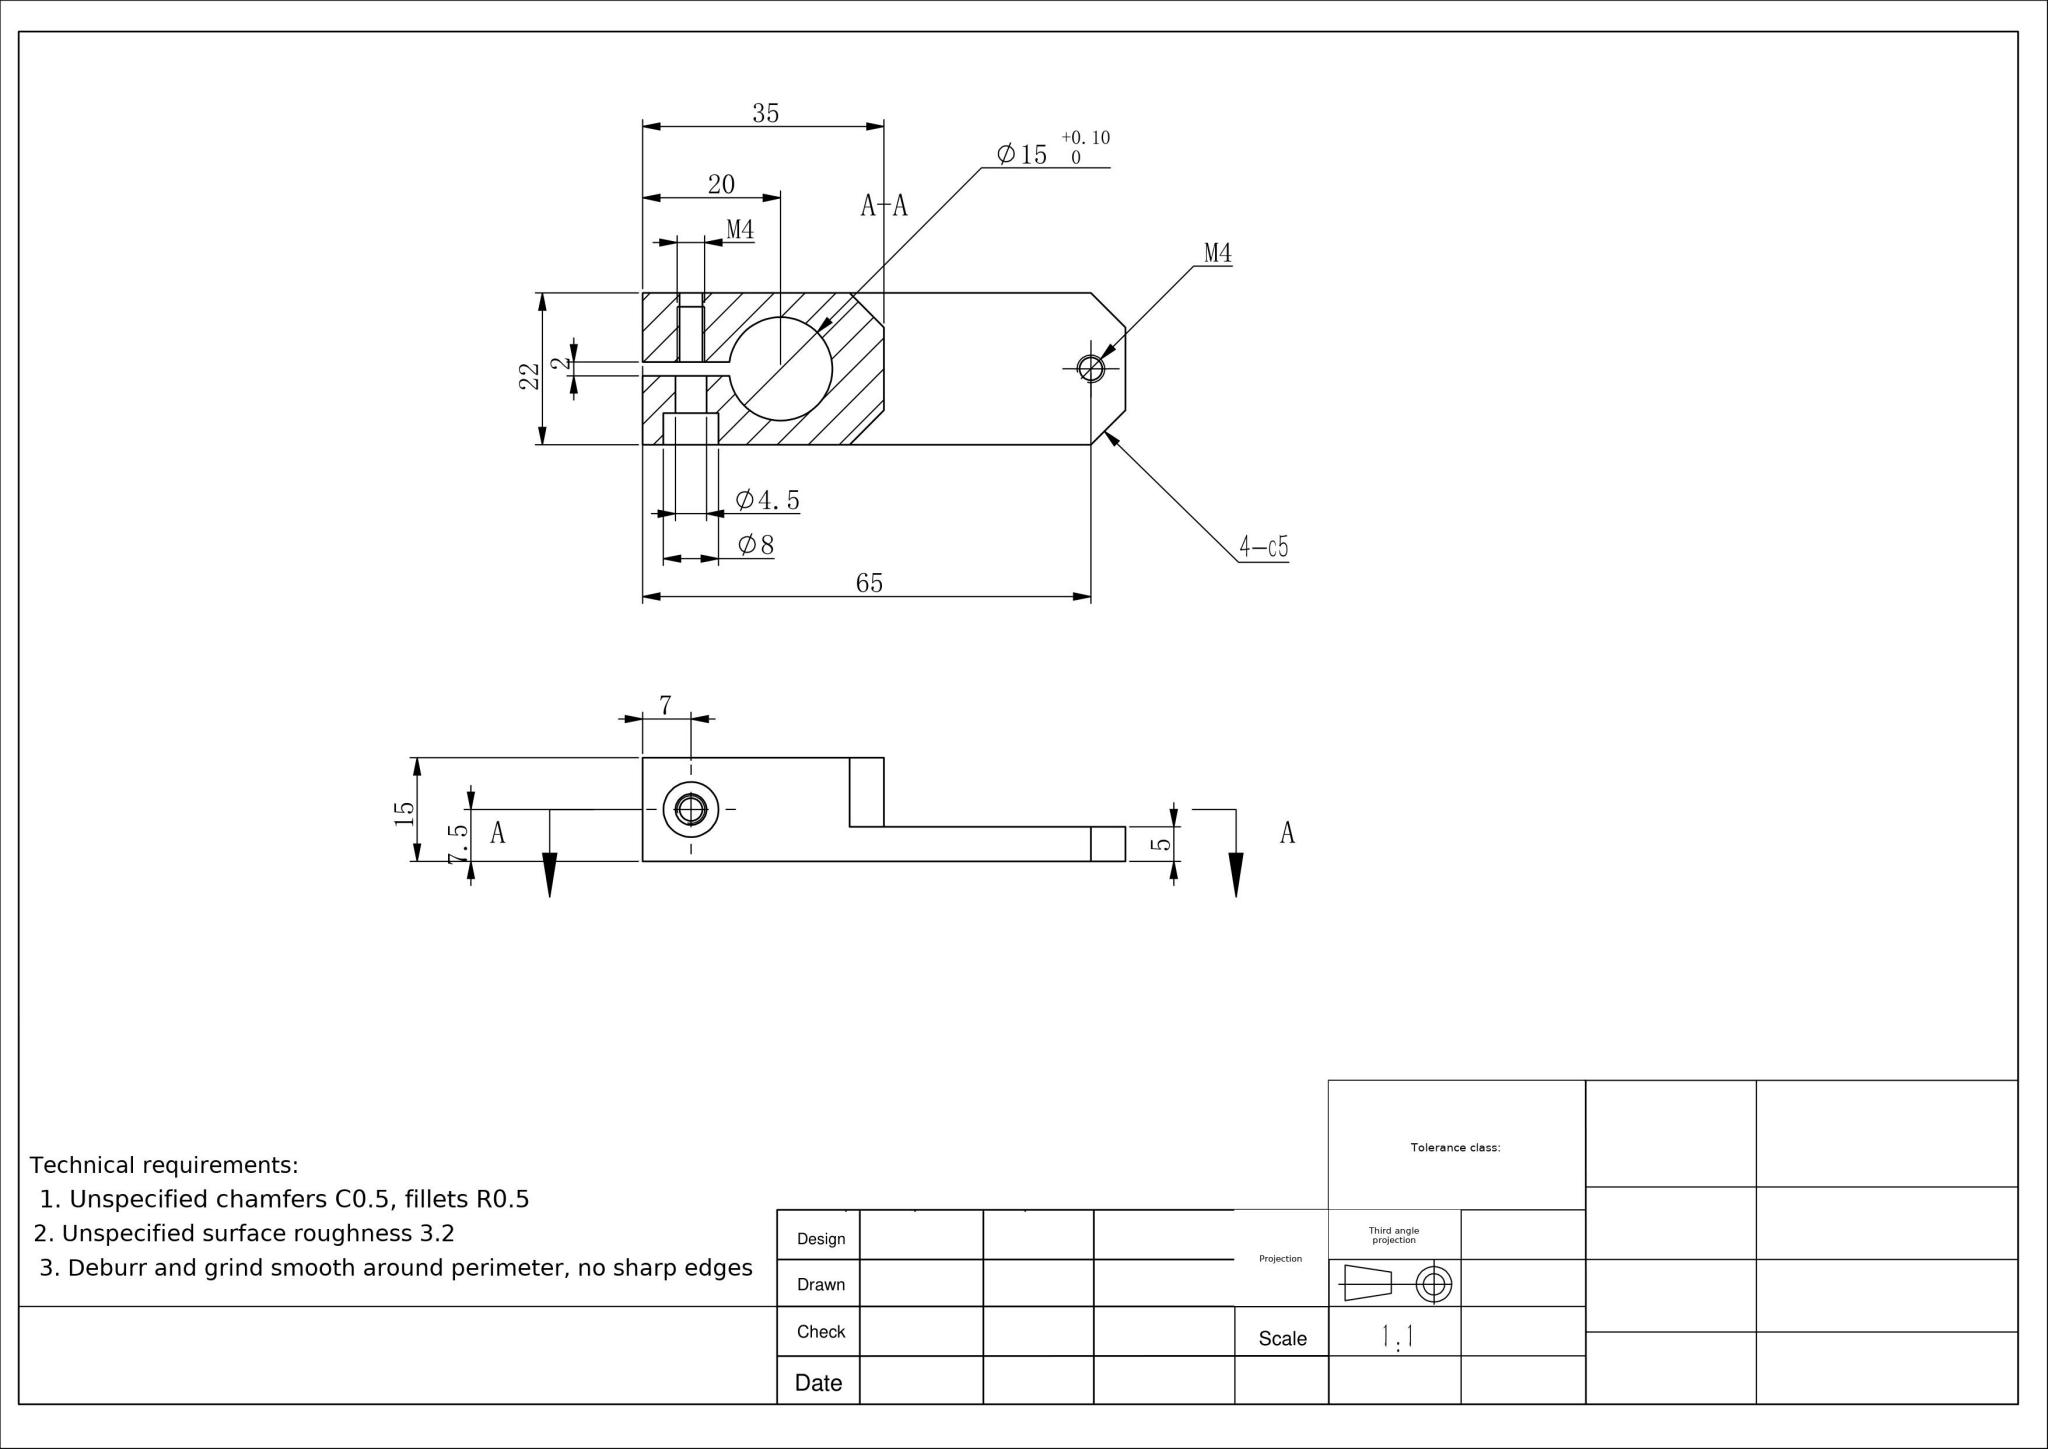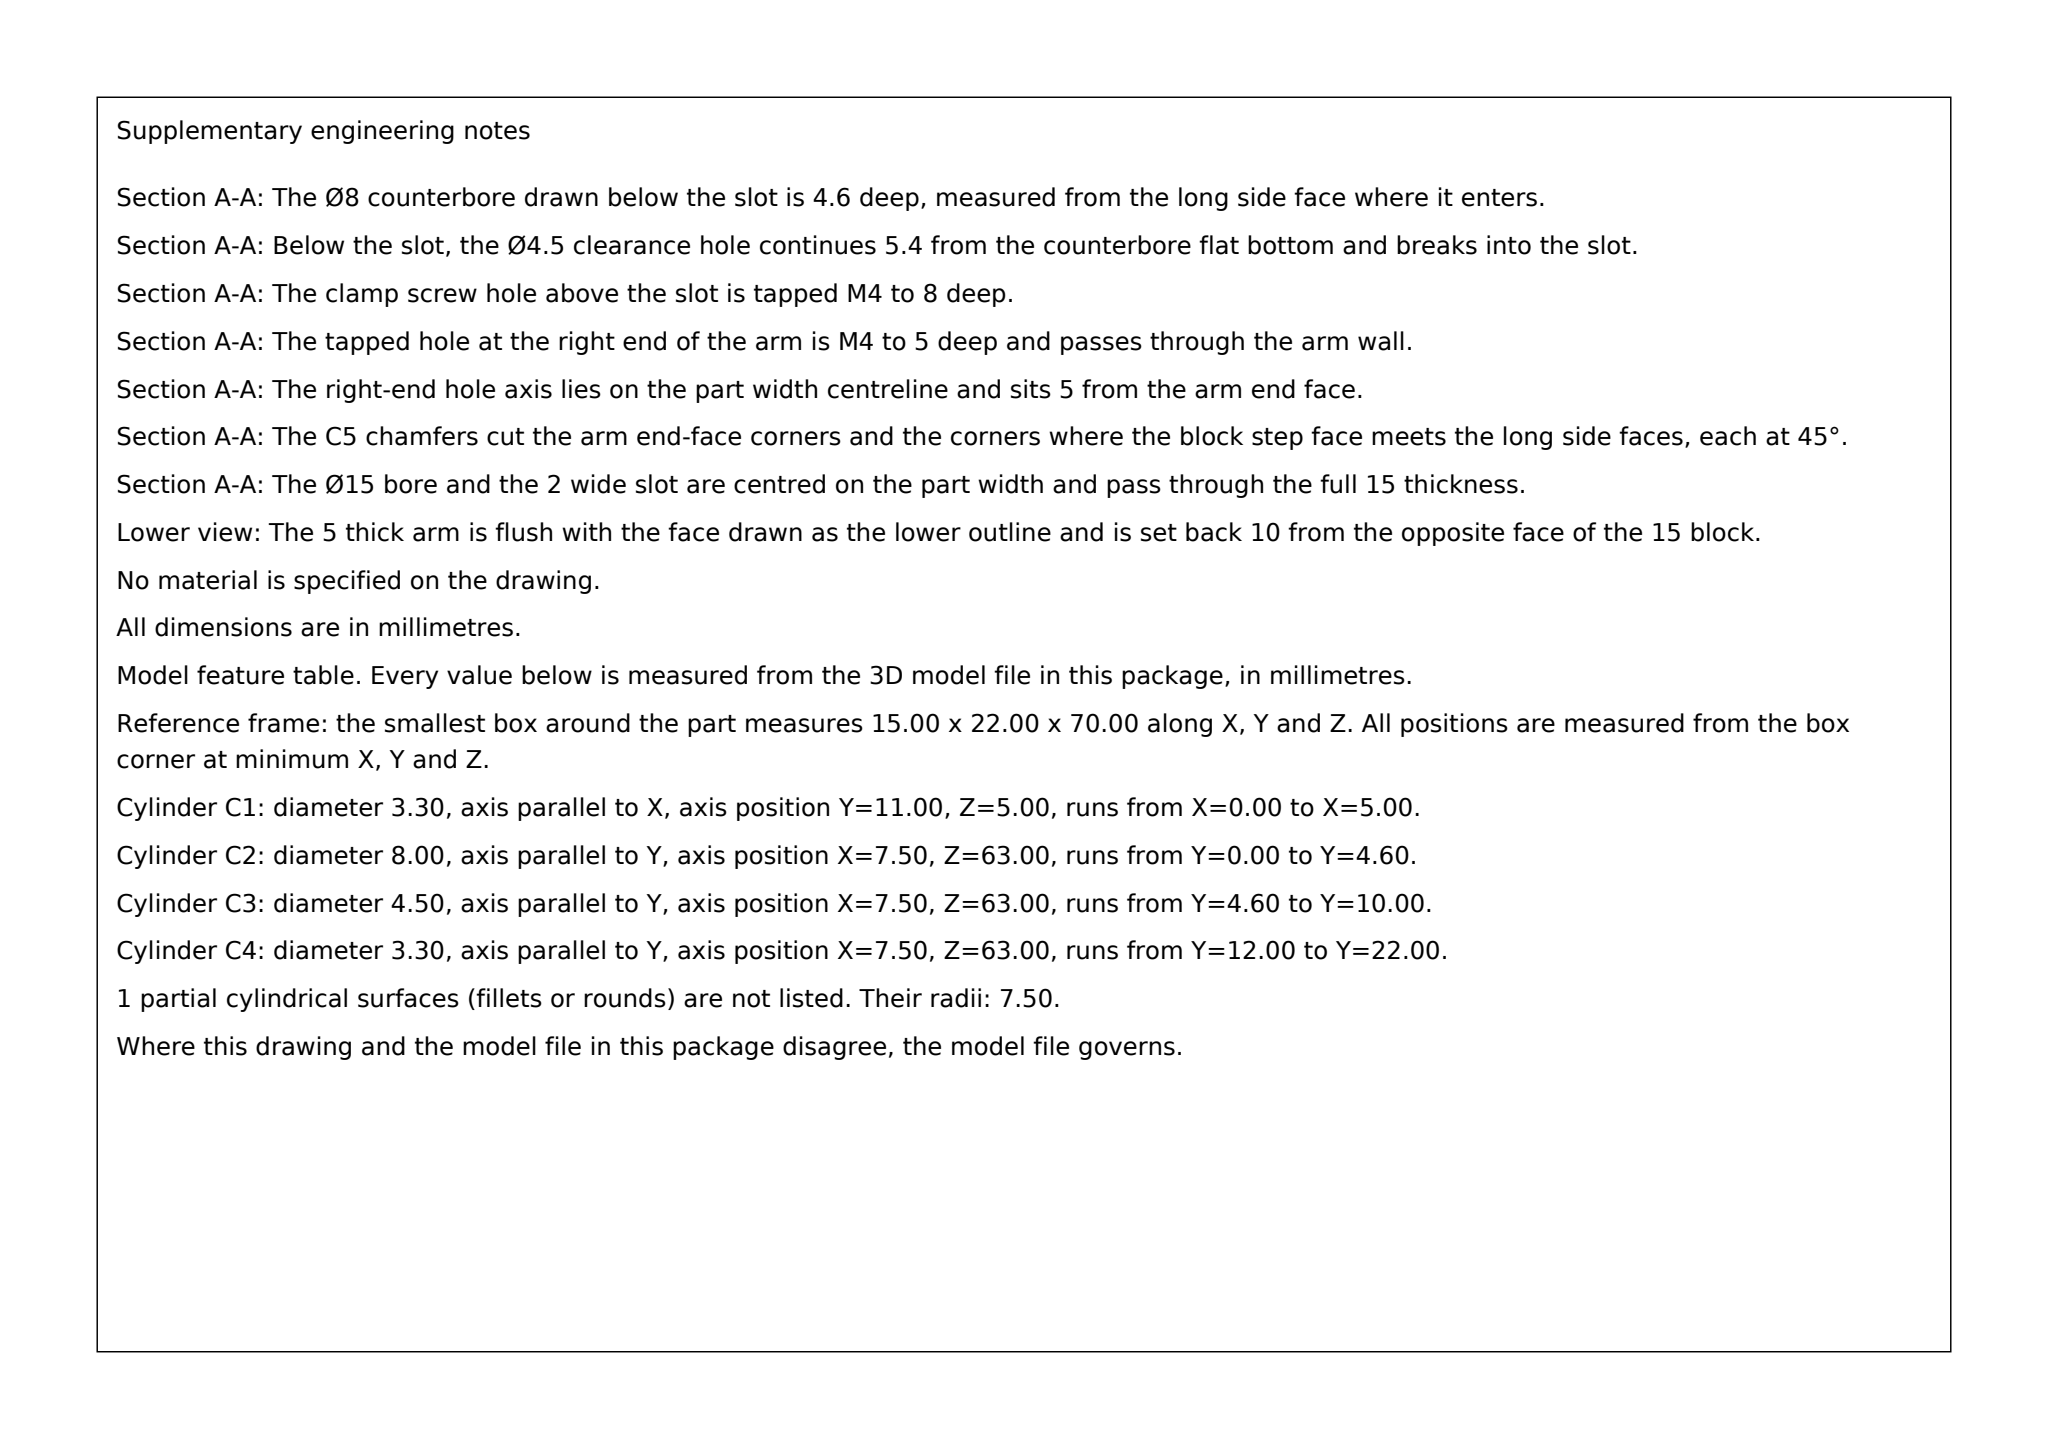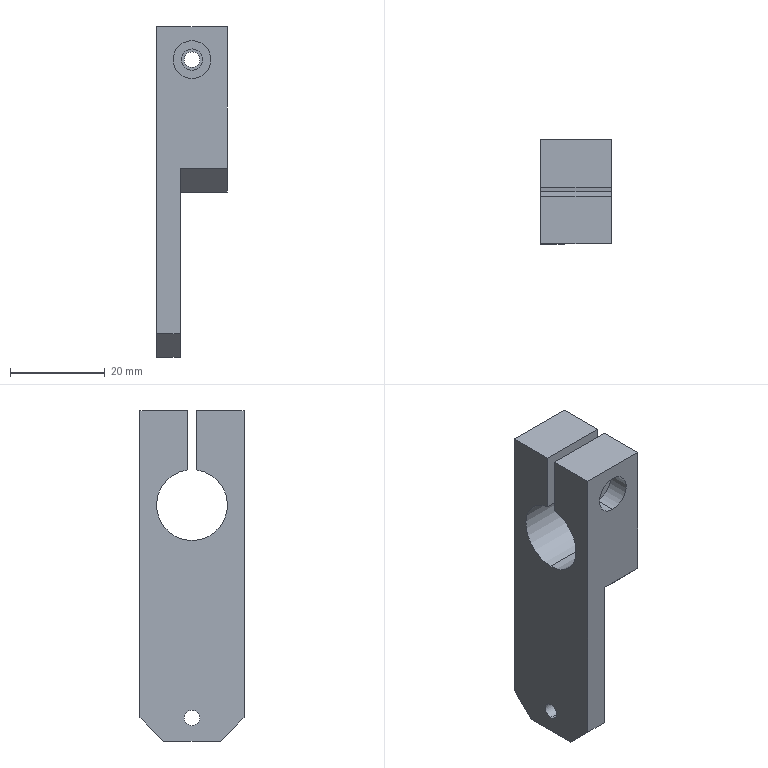Part | SolidWorks | mm | 1 solid | 26 faces | box 15 x 22 x 70 mm | volume 11553 mm3 | plane 16 | cylinder 10 | commonest cylinder face diameters 3.3 x4 8 x2 4.5 x2 15 x2
Drawing notes:
OVERALL LG 70 (END FACE 5 BEYOND END M4 AXIS) | from the solid: bbox_xyz z=70; M4 (Ø3.3 x-axis) at z=5, so 70-5=65 matches given dim
Ø15 +0.10/0 BORE AXIS 11 FROM BOTTOM FACE OF 22 | from the solid: cylinder [15.0,'x',[null,11.0,50.0],15.0] -> y=11 of 22 high bbox
2 WIDE SLOT CL ON Ø15 BORE AXIS, 11 FROM BOTTOM FACE | from the solid: y planes at 10.0 and 12.0 -> 2 wide slot centred y=11 = bore axis y
END M4 THRU IN 5 THK TONGUE: AXIS 11 FROM BOTTOM FACE | from the solid: cylinder [3.3,'x',[null,11.0,5.0],5.0]; x planes 0 and 5 = 5 thk tongue
END M4 AXIS 5 FROM END FACE | from the solid: cylinder [3.3,'x',[null,11.0,5.0]] vs bbox z=0 end face
build123d program:
from build123d import *

# Parameters (mm, degrees)
SKETCH1_W                                            = 70
SKETCH1_H                                            = 22
BOSS_EXTRUDE1_DEPTH                                  = 15
SKETCH2_R                                            = 7.5
CUT_EXTRUDE1_DEPTH                                   = 40.636
SKETCH3_W                                            = 29.611
SKETCH3_H                                            = 2
CUT_EXTRUDE2_DEPTH                                   = 40.636
HOLE_SIZE_ACCORDING_TO_THE_TYPE_OF_HEXAG_D           = 4.5
HOLE_SIZE_ACCORDING_TO_THE_TYPE_OF_HEXAG_DEPTH       = 10
HOLE_SIZE_ACCORDING_TO_THE_TYPE_OF_HEXAG_CBORE_D     = 8
HOLE_SIZE_ACCORDING_TO_THE_TYPE_OF_HEXAG_CBORE_DEPTH = 4.6
M4_TAPPED_HOLE1_D                                    = 3.3
M4_TAPPED_HOLE1_DEPTH                                = 11.5
M4_TAPPED_HOLE1_TIP                                  = 0.9914
SKETCH8_W                                            = 35
SKETCH8_H                                            = 22
CUT_EXTRUDE3_DEPTH                                   = 10
CHAMFER1_SIZE                                        = 5
M4_TAPPED_HOLE2_D                                    = 3.3
CHAMFER2_SIZE                                        = 5


with BuildPart() as part:
    # Sketch1 → Boss-Extrude1 (new body)
    with BuildSketch(Plane(origin=(0, 0, 0), x_dir=(0, 0, -1), z_dir=(1, 0, 0))):
        Rectangle(SKETCH1_W, SKETCH1_H)
    extrude(amount=BOSS_EXTRUDE1_DEPTH)

    # Sketch2 → Cut-Extrude1 (cut, through all)
    with BuildSketch(Plane(origin=(15, 0, 0), x_dir=(0, 0, -1), z_dir=(1, 0, 0))):
        with Locations((-15, 0)):
            Circle(SKETCH2_R)
    extrude(amount=-CUT_EXTRUDE1_DEPTH, mode=Mode.SUBTRACT)

    # Sketch3 → Cut-Extrude2 (cut, through all)
    with BuildSketch(Plane(origin=(15, 0, 0), x_dir=(0, 0, -1), z_dir=(1, 0, 0))):
        with Locations((-35, 0)):
            Rectangle(SKETCH3_W, SKETCH3_H)
    extrude(amount=-CUT_EXTRUDE2_DEPTH, mode=Mode.SUBTRACT)

    # Hole size according to the type of hexag
    with Locations(Plane(origin=(0, -11, 0), x_dir=(-1, 0, 0), z_dir=(0, -1, 0))):
        with Locations((-7.5, -28)):
            CounterBoreHole(HOLE_SIZE_ACCORDING_TO_THE_TYPE_OF_HEXAG_D / 2, HOLE_SIZE_ACCORDING_TO_THE_TYPE_OF_HEXAG_CBORE_D / 2, HOLE_SIZE_ACCORDING_TO_THE_TYPE_OF_HEXAG_CBORE_DEPTH, depth=HOLE_SIZE_ACCORDING_TO_THE_TYPE_OF_HEXAG_DEPTH)

    # M4 Tapped Hole1
    with Locations(Plane(origin=(0, 1, 0), x_dir=(-1, 0, 0), z_dir=(0, -1, 0))):
        with Locations((-7.5, -28)):
            Hole(M4_TAPPED_HOLE1_D / 2, depth=M4_TAPPED_HOLE1_DEPTH)
            with Locations((0, 0, -(M4_TAPPED_HOLE1_DEPTH + M4_TAPPED_HOLE1_TIP / 2))):  # 118° drill point
                Cone(0, M4_TAPPED_HOLE1_D / 2, M4_TAPPED_HOLE1_TIP, mode=Mode.SUBTRACT)

    # Sketch8 → Cut-Extrude3 (cut)
    with BuildSketch(Plane(origin=(15, 0, 0), x_dir=(0, 0, -1), z_dir=(1, 0, 0))):
        with Locations((17.5, 0)):
            Rectangle(SKETCH8_W, SKETCH8_H)
    extrude(amount=-CUT_EXTRUDE3_DEPTH, mode=Mode.SUBTRACT)

    # Chamfer1
    chamfer1_edges = [part.edges().sort_by_distance(p)[0] for p in [
        (2.5, 11, -35),
        (2.5, -11, -35),
    ]]
    chamfer(chamfer1_edges, length=CHAMFER1_SIZE)

    # M4 Tapped Hole2 (through all)
    with Locations(Plane(origin=(5, 0, 0), x_dir=(0, 0, -1), z_dir=(1, 0, 0))):
        with Locations((30, 0)):
            Hole(M4_TAPPED_HOLE2_D / 2)

    # Chamfer2
    chamfer2_edges = [part.edges().sort_by_distance(p)[0] for p in [
        (10, -11, 0),
        (10, 11, 0),
    ]]
    chamfer(chamfer2_edges, length=CHAMFER2_SIZE)


solid = part.part
STEP:
#1=CARTESIAN_POINT('',(0.,-0.,-28.35));
#2=VERTEX_POINT('',#1);
#3=CARTESIAN_POINT('',(0.,-0.,-31.65));
#4=VERTEX_POINT('',#3);
#5=CARTESIAN_POINT('',(0.,-0.,-30.));
#6=DIRECTION('',(1.,0.,0.));
#7=DIRECTION('',(0.,0.,-1.));
#8=AXIS2_PLACEMENT_3D('',#5,#6,#7);
#9=CIRCLE('',#8,1.65);
#10=EDGE_CURVE('',#2,#4,#9,.T.);
#11=ORIENTED_EDGE('',*,*,#10,.F.);
#12=CARTESIAN_POINT('',(5.,-0.,-28.35));
#13=VERTEX_POINT('',#12);
#14=CARTESIAN_POINT('',(5.,-0.,-28.35));
#15=DIRECTION('',(1.,0.,0.));
#16=VECTOR('',#15,1000.);
#17=LINE('',#14,#16);
#18=EDGE_CURVE('',#2,#13,#17,.T.);
#19=ORIENTED_EDGE('',*,*,#18,.T.);
#20=CARTESIAN_POINT('',(5.,-0.,-31.65));
#21=VERTEX_POINT('',#20);
#22=CARTESIAN_POINT('',(5.,-0.,-30.));
#23=DIRECTION('',(1.,0.,0.));
#24=DIRECTION('',(0.,0.,-1.));
#25=AXIS2_PLACEMENT_3D('',#22,#23,#24);
#26=CIRCLE('',#25,1.65);
#27=EDGE_CURVE('',#13,#21,#26,.T.);
#28=ORIENTED_EDGE('',*,*,#27,.T.);
#29=CARTESIAN_POINT('',(5.,-0.,-31.65));
#30=DIRECTION('',(1.,0.,0.));
#31=VECTOR('',#30,1000.);
#32=LINE('',#29,#31);
#33=EDGE_CURVE('',#4,#21,#32,.T.);
#34=ORIENTED_EDGE('',*,*,#33,.F.);
#35=EDGE_LOOP('',(#11,#19,#28,#34));
#36=FACE_OUTER_BOUND('',#35,.T.);
#37=CARTESIAN_POINT('',(5.,-0.,-30.));
#38=DIRECTION('',(1.,0.,0.));
#39=DIRECTION('',(0.,0.,-1.));
#40=AXIS2_PLACEMENT_3D('',#37,#38,#39);
#41=CYLINDRICAL_SURFACE('',#40,1.65);
#42=ADVANCED_FACE('',(#36),#41,.F.);
#43=CARTESIAN_POINT('',(7.5,11.,29.65));
#44=VERTEX_POINT('',#43);
#45=CARTESIAN_POINT('',(7.5,11.,26.35));
#46=VERTEX_POINT('',#45);
#47=CARTESIAN_POINT('',(7.5,11.,28.));
#48=DIRECTION('',(0.,-1.,0.));
#49=DIRECTION('',(0.,0.,-1.));
#50=AXIS2_PLACEMENT_3D('',#47,#48,#49);
#51=CIRCLE('',#50,1.65);
#52=EDGE_CURVE('',#44,#46,#51,.T.);
#53=ORIENTED_EDGE('',*,*,#52,.F.);
#54=CARTESIAN_POINT('',(7.5,1.,29.65));
#55=VERTEX_POINT('',#54);
#56=CARTESIAN_POINT('',(7.5,1.,29.65));
#57=DIRECTION('',(0.,-1.,0.));
#58=VECTOR('',#57,1000.);
#59=LINE('',#56,#58);
#60=EDGE_CURVE('',#44,#55,#59,.T.);
#61=ORIENTED_EDGE('',*,*,#60,.T.);
#62=CARTESIAN_POINT('',(7.5,1.,26.35));
#63=VERTEX_POINT('',#62);
#64=CARTESIAN_POINT('',(7.5,1.,28.));
#65=DIRECTION('',(0.,-1.,0.));
#66=DIRECTION('',(0.,0.,-1.));
#67=AXIS2_PLACEMENT_3D('',#64,#65,#66);
#68=CIRCLE('',#67,1.65);
#69=EDGE_CURVE('',#55,#63,#68,.T.);
#70=ORIENTED_EDGE('',*,*,#69,.T.);
#71=CARTESIAN_POINT('',(7.5,1.,26.35));
#72=DIRECTION('',(0.,-1.,0.));
#73=VECTOR('',#72,1000.);
#74=LINE('',#71,#73);
#75=EDGE_CURVE('',#46,#63,#74,.T.);
#76=ORIENTED_EDGE('',*,*,#75,.F.);
#77=EDGE_LOOP('',(#53,#61,#70,#76));
#78=FACE_OUTER_BOUND('',#77,.T.);
#79=CARTESIAN_POINT('',(7.5,1.,28.));
#80=DIRECTION('',(0.,-1.,0.));
#81=DIRECTION('',(0.,0.,-1.));
#82=AXIS2_PLACEMENT_3D('',#79,#80,#81);
#83=CYLINDRICAL_SURFACE('',#82,1.65);
#84=ADVANCED_FACE('',(#78),#83,.F.);
#85=CARTESIAN_POINT('',(7.5,-6.4,32.));
#86=VERTEX_POINT('',#85);
#87=CARTESIAN_POINT('',(7.5,-6.4,24.));
#88=VERTEX_POINT('',#87);
#89=CARTESIAN_POINT('',(7.5,-6.4,28.));
#90=DIRECTION('',(0.,-1.,0.));
#91=DIRECTION('',(0.,0.,-1.));
#92=AXIS2_PLACEMENT_3D('',#89,#90,#91);
#93=CIRCLE('',#92,4.);
#94=EDGE_CURVE('',#86,#88,#93,.T.);
#95=ORIENTED_EDGE('',*,*,#94,.F.);
#96=CARTESIAN_POINT('',(7.5,-11.,32.));
#97=VERTEX_POINT('',#96);
#98=CARTESIAN_POINT('',(7.5,-11.,32.));
#99=DIRECTION('',(0.,-1.,0.));
#100=VECTOR('',#99,1000.);
#101=LINE('',#98,#100);
#102=EDGE_CURVE('',#86,#97,#101,.T.);
#103=ORIENTED_EDGE('',*,*,#102,.T.);
#104=CARTESIAN_POINT('',(7.5,-11.,24.));
#105=VERTEX_POINT('',#104);
#106=CARTESIAN_POINT('',(7.5,-11.,28.));
#107=DIRECTION('',(0.,-1.,0.));
#108=DIRECTION('',(0.,0.,-1.));
#109=AXIS2_PLACEMENT_3D('',#106,#107,#108);
#110=CIRCLE('',#109,4.);
#111=EDGE_CURVE('',#97,#105,#110,.T.);
#112=ORIENTED_EDGE('',*,*,#111,.T.);
#113=CARTESIAN_POINT('',(7.5,-11.,24.));
#114=DIRECTION('',(0.,-1.,0.));
#115=VECTOR('',#114,1000.);
#116=LINE('',#113,#115);
#117=EDGE_CURVE('',#88,#105,#116,.T.);
#118=ORIENTED_EDGE('',*,*,#117,.F.);
#119=EDGE_LOOP('',(#95,#103,#112,#118));
#120=FACE_OUTER_BOUND('',#119,.T.);
#121=CARTESIAN_POINT('',(7.5,-11.,28.));
#122=DIRECTION('',(0.,-1.,0.));
#123=DIRECTION('',(0.,0.,-1.));
#124=AXIS2_PLACEMENT_3D('',#121,#122,#123);
#125=CYLINDRICAL_SURFACE('',#124,4.);
#126=ADVANCED_FACE('',(#120),#125,.F.);
#127=CARTESIAN_POINT('',(7.5,-1.,30.25));
#128=VERTEX_POINT('',#127);
#129=CARTESIAN_POINT('',(7.5,-1.,25.75));
#130=VERTEX_POINT('',#129);
#131=CARTESIAN_POINT('',(7.5,-1.,28.));
#132=DIRECTION('',(0.,-1.,0.));
#133=DIRECTION('',(0.,0.,-1.));
#134=AXIS2_PLACEMENT_3D('',#131,#132,#133);
#135=CIRCLE('',#134,2.25);
#136=EDGE_CURVE('',#128,#130,#135,.T.);
#137=ORIENTED_EDGE('',*,*,#136,.F.);
#138=CARTESIAN_POINT('',(7.5,-6.4,30.25));
#139=VERTEX_POINT('',#138);
#140=CARTESIAN_POINT('',(7.5,-11.,30.25));
#141=DIRECTION('',(0.,-1.,0.));
#142=VECTOR('',#141,1000.);
#143=LINE('',#140,#142);
#144=EDGE_CURVE('',#128,#139,#143,.T.);
#145=ORIENTED_EDGE('',*,*,#144,.T.);
#146=CARTESIAN_POINT('',(7.5,-6.4,25.75));
#147=VERTEX_POINT('',#146);
#148=CARTESIAN_POINT('',(7.5,-6.4,28.));
#149=DIRECTION('',(0.,-1.,0.));
#150=DIRECTION('',(0.,0.,-1.));
#151=AXIS2_PLACEMENT_3D('',#148,#149,#150);
#152=CIRCLE('',#151,2.25);
#153=EDGE_CURVE('',#139,#147,#152,.T.);
#154=ORIENTED_EDGE('',*,*,#153,.T.);
#155=CARTESIAN_POINT('',(7.5,-11.,25.75));
#156=DIRECTION('',(0.,-1.,0.));
#157=VECTOR('',#156,1000.);
#158=LINE('',#155,#157);
#159=EDGE_CURVE('',#130,#147,#158,.T.);
#160=ORIENTED_EDGE('',*,*,#159,.F.);
#161=EDGE_LOOP('',(#137,#145,#154,#160));
#162=FACE_OUTER_BOUND('',#161,.T.);
#163=CARTESIAN_POINT('',(7.5,-11.,28.));
#164=DIRECTION('',(0.,-1.,0.));
#165=DIRECTION('',(0.,0.,-1.));
#166=AXIS2_PLACEMENT_3D('',#163,#164,#165);
#167=CYLINDRICAL_SURFACE('',#166,2.25);
#168=ADVANCED_FACE('',(#162),#167,.F.);
#169=CARTESIAN_POINT('',(0.,0.,7.5));
#170=VERTEX_POINT('',#169);
#171=CARTESIAN_POINT('',(0.,1.,22.433));
#172=VERTEX_POINT('',#171);
#173=CARTESIAN_POINT('',(0.,0.,15.));
#174=DIRECTION('',(1.,0.,0.));
#175=DIRECTION('',(0.,0.,-1.));
#176=AXIS2_PLACEMENT_3D('',#173,#174,#175);
#177=CIRCLE('',#176,7.5);
#178=EDGE_CURVE('',#170,#172,#177,.T.);
#179=ORIENTED_EDGE('',*,*,#178,.F.);
#180=CARTESIAN_POINT('',(15.,0.,7.5));
#181=VERTEX_POINT('',#180);
#182=CARTESIAN_POINT('',(0.,0.,7.5));
#183=DIRECTION('',(1.,0.,0.));
#184=VECTOR('',#183,1000.);
#185=LINE('',#182,#184);
#186=EDGE_CURVE('',#170,#181,#185,.T.);
#187=ORIENTED_EDGE('',*,*,#186,.T.);
#188=CARTESIAN_POINT('',(15.,1.,22.433));
#189=VERTEX_POINT('',#188);
#190=CARTESIAN_POINT('',(15.,0.,15.));
#191=DIRECTION('',(1.,0.,0.));
#192=DIRECTION('',(0.,0.,-1.));
#193=AXIS2_PLACEMENT_3D('',#190,#191,#192);
#194=CIRCLE('',#193,7.5);
#195=EDGE_CURVE('',#181,#189,#194,.T.);
#196=ORIENTED_EDGE('',*,*,#195,.T.);
#197=CARTESIAN_POINT('',(0.,1.,22.433));
#198=DIRECTION('',(-1.,0.,0.));
#199=VECTOR('',#198,1000.);
#200=LINE('',#197,#199);
#201=EDGE_CURVE('',#189,#172,#200,.T.);
#202=ORIENTED_EDGE('',*,*,#201,.T.);
#203=EDGE_LOOP('',(#179,#187,#196,#202));
#204=FACE_OUTER_BOUND('',#203,.T.);
#205=CARTESIAN_POINT('',(0.,0.,15.));
#206=DIRECTION('',(1.,0.,0.));
#207=DIRECTION('',(0.,0.,-1.));
#208=AXIS2_PLACEMENT_3D('',#205,#206,#207);
#209=CYLINDRICAL_SURFACE('',#208,7.5);
#210=ADVANCED_FACE('',(#204),#209,.F.);
#211=CARTESIAN_POINT('',(5.,-11.,5.));
#212=VERTEX_POINT('',#211);
#213=CARTESIAN_POINT('',(5.,-11.,-30.));
#214=VERTEX_POINT('',#213);
#215=CARTESIAN_POINT('',(5.,-11.,-35.));
#216=DIRECTION('',(0.,0.,-1.));
#217=VECTOR('',#216,1000.);
#218=LINE('',#215,#217);
#219=EDGE_CURVE('',#212,#214,#218,.T.);
#220=ORIENTED_EDGE('',*,*,#219,.F.);
#221=CARTESIAN_POINT('',(15.,-11.,5.));
#222=VERTEX_POINT('',#221);
#223=CARTESIAN_POINT('',(15.,-11.,5.));
#224=DIRECTION('',(1.,0.,0.));
#225=VECTOR('',#224,1000.);
#226=LINE('',#223,#225);
#227=EDGE_CURVE('',#212,#222,#226,.T.);
#228=ORIENTED_EDGE('',*,*,#227,.T.);
#229=CARTESIAN_POINT('',(15.,-11.,35.));
#230=VERTEX_POINT('',#229);
#231=CARTESIAN_POINT('',(15.,-11.,35.));
#232=DIRECTION('',(0.,0.,-1.));
#233=VECTOR('',#232,1000.);
#234=LINE('',#231,#233);
#235=EDGE_CURVE('',#230,#222,#234,.T.);
#236=ORIENTED_EDGE('',*,*,#235,.F.);
#237=CARTESIAN_POINT('',(0.,-11.,35.));
#238=VERTEX_POINT('',#237);
#239=CARTESIAN_POINT('',(15.,-11.,35.));
#240=DIRECTION('',(-1.,0.,0.));
#241=VECTOR('',#240,1000.);
#242=LINE('',#239,#241);
#243=EDGE_CURVE('',#230,#238,#242,.T.);
#244=ORIENTED_EDGE('',*,*,#243,.T.);
#245=CARTESIAN_POINT('',(0.,-11.,-30.));
#246=VERTEX_POINT('',#245);
#247=CARTESIAN_POINT('',(0.,-11.,35.));
#248=DIRECTION('',(0.,0.,-1.));
#249=VECTOR('',#248,1000.);
#250=LINE('',#247,#249);
#251=EDGE_CURVE('',#238,#246,#250,.T.);
#252=ORIENTED_EDGE('',*,*,#251,.T.);
#253=CARTESIAN_POINT('',(15.,-11.,-30.));
#254=DIRECTION('',(1.,0.,0.));
#255=VECTOR('',#254,1000.);
#256=LINE('',#253,#255);
#257=EDGE_CURVE('',#246,#214,#256,.T.);
#258=ORIENTED_EDGE('',*,*,#257,.T.);
#259=EDGE_LOOP('',(#220,#228,#236,#244,#252,#258));
#260=FACE_OUTER_BOUND('',#259,.T.);
#261=CARTESIAN_POINT('',(7.5,-11.,28.));
#262=DIRECTION('',(0.,-1.,0.));
#263=DIRECTION('',(0.,0.,-1.));
#264=AXIS2_PLACEMENT_3D('',#261,#262,#263);
#265=CIRCLE('',#264,4.);
#266=EDGE_CURVE('',#105,#97,#265,.T.);
#267=ORIENTED_EDGE('',*,*,#266,.F.);
#268=ORIENTED_EDGE('',*,*,#111,.F.);
#269=EDGE_LOOP('',(#267,#268));
#270=FACE_BOUND('',#269,.T.);
#271=CARTESIAN_POINT('',(15.,-11.,35.));
#272=DIRECTION('',(0.,1.,0.));
#273=DIRECTION('',(0.,0.,1.));
#274=AXIS2_PLACEMENT_3D('',#271,#272,#273);
#275=PLANE('',#274);
#276=ADVANCED_FACE('',(#260,#270),#275,.F.);
#277=CARTESIAN_POINT('',(15.,-1.,35.));
#278=VERTEX_POINT('',#277);
#279=CARTESIAN_POINT('',(15.,-11.,35.));
#280=DIRECTION('',(0.,-1.,0.));
#281=VECTOR('',#280,1000.);
#282=LINE('',#279,#281);
#283=EDGE_CURVE('',#278,#230,#282,.T.);
#284=ORIENTED_EDGE('',*,*,#283,.F.);
#285=CARTESIAN_POINT('',(0.,-1.,35.));
#286=VERTEX_POINT('',#285);
#287=CARTESIAN_POINT('',(15.,-1.,35.));
#288=DIRECTION('',(-1.,0.,0.));
#289=VECTOR('',#288,1000.);
#290=LINE('',#287,#289);
#291=EDGE_CURVE('',#278,#286,#290,.T.);
#292=ORIENTED_EDGE('',*,*,#291,.T.);
#293=CARTESIAN_POINT('',(0.,-11.,35.));
#294=DIRECTION('',(0.,-1.,0.));
#295=VECTOR('',#294,1000.);
#296=LINE('',#293,#295);
#297=EDGE_CURVE('',#286,#238,#296,.T.);
#298=ORIENTED_EDGE('',*,*,#297,.T.);
#299=ORIENTED_EDGE('',*,*,#243,.F.);
#300=EDGE_LOOP('',(#284,#292,#298,#299));
#301=FACE_OUTER_BOUND('',#300,.T.);
#302=CARTESIAN_POINT('',(15.,-11.,35.));
#303=DIRECTION('',(0.,0.,-1.));
#304=DIRECTION('',(-1.,0.,0.));
#305=AXIS2_PLACEMENT_3D('',#302,#303,#304);
#306=PLANE('',#305);
#307=ADVANCED_FACE('',(#301),#306,.F.);
#308=CARTESIAN_POINT('',(5.,-6.,-35.));
#309=VERTEX_POINT('',#308);
#310=CARTESIAN_POINT('',(5.,6.,-35.));
#311=VERTEX_POINT('',#310);
#312=CARTESIAN_POINT('',(5.,11.,-35.));
#313=DIRECTION('',(0.,1.,0.));
#314=VECTOR('',#313,1000.);
#315=LINE('',#312,#314);
#316=EDGE_CURVE('',#309,#311,#315,.T.);
#317=ORIENTED_EDGE('',*,*,#316,.F.);
#318=CARTESIAN_POINT('',(0.,-6.,-35.));
#319=VERTEX_POINT('',#318);
#320=CARTESIAN_POINT('',(15.,-6.,-35.));
#321=DIRECTION('',(-1.,0.,0.));
#322=VECTOR('',#321,1000.);
#323=LINE('',#320,#322);
#324=EDGE_CURVE('',#309,#319,#323,.T.);
#325=ORIENTED_EDGE('',*,*,#324,.T.);
#326=CARTESIAN_POINT('',(0.,6.,-35.));
#327=VERTEX_POINT('',#326);
#328=CARTESIAN_POINT('',(0.,-11.,-35.));
#329=DIRECTION('',(0.,1.,0.));
#330=VECTOR('',#329,1000.);
#331=LINE('',#328,#330);
#332=EDGE_CURVE('',#319,#327,#331,.T.);
#333=ORIENTED_EDGE('',*,*,#332,.T.);
#334=CARTESIAN_POINT('',(15.,6.,-35.));
#335=DIRECTION('',(1.,0.,0.));
#336=VECTOR('',#335,1000.);
#337=LINE('',#334,#336);
#338=EDGE_CURVE('',#327,#311,#337,.T.);
#339=ORIENTED_EDGE('',*,*,#338,.T.);
#340=EDGE_LOOP('',(#317,#325,#333,#339));
#341=FACE_OUTER_BOUND('',#340,.T.);
#342=CARTESIAN_POINT('',(15.,-11.,-35.));
#343=DIRECTION('',(0.,0.,1.));
#344=DIRECTION('',(1.,0.,0.));
#345=AXIS2_PLACEMENT_3D('',#342,#343,#344);
#346=PLANE('',#345);
#347=ADVANCED_FACE('',(#341),#346,.F.);
#348=CARTESIAN_POINT('',(7.5,11.,28.));
#349=DIRECTION('',(0.,-1.,0.));
#350=DIRECTION('',(0.,0.,-1.));
#351=AXIS2_PLACEMENT_3D('',#348,#349,#350);
#352=CIRCLE('',#351,1.65);
#353=EDGE_CURVE('',#46,#44,#352,.T.);
#354=ORIENTED_EDGE('',*,*,#353,.T.);
#355=ORIENTED_EDGE('',*,*,#52,.T.);
#356=EDGE_LOOP('',(#354,#355));
#357=FACE_BOUND('',#356,.T.);
#358=CARTESIAN_POINT('',(15.,11.,5.));
#359=VERTEX_POINT('',#358);
#360=CARTESIAN_POINT('',(15.,11.,35.));
#361=VERTEX_POINT('',#360);
#362=CARTESIAN_POINT('',(15.,11.,35.));
#363=DIRECTION('',(0.,0.,1.));
#364=VECTOR('',#363,1000.);
#365=LINE('',#362,#364);
#366=EDGE_CURVE('',#359,#361,#365,.T.);
#367=ORIENTED_EDGE('',*,*,#366,.F.);
#368=CARTESIAN_POINT('',(5.,11.,5.));
#369=VERTEX_POINT('',#368);
#370=CARTESIAN_POINT('',(15.,11.,5.));
#371=DIRECTION('',(-1.,0.,0.));
#372=VECTOR('',#371,1000.);
#373=LINE('',#370,#372);
#374=EDGE_CURVE('',#359,#369,#373,.T.);
#375=ORIENTED_EDGE('',*,*,#374,.T.);
#376=CARTESIAN_POINT('',(5.,11.,-30.));
#377=VERTEX_POINT('',#376);
#378=CARTESIAN_POINT('',(5.,11.,-35.));
#379=DIRECTION('',(0.,0.,1.));
#380=VECTOR('',#379,1000.);
#381=LINE('',#378,#380);
#382=EDGE_CURVE('',#377,#369,#381,.T.);
#383=ORIENTED_EDGE('',*,*,#382,.F.);
#384=CARTESIAN_POINT('',(0.,11.,-30.));
#385=VERTEX_POINT('',#384);
#386=CARTESIAN_POINT('',(15.,11.,-30.));
#387=DIRECTION('',(-1.,0.,0.));
#388=VECTOR('',#387,1000.);
#389=LINE('',#386,#388);
#390=EDGE_CURVE('',#377,#385,#389,.T.);
#391=ORIENTED_EDGE('',*,*,#390,.T.);
#392=CARTESIAN_POINT('',(0.,11.,35.));
#393=VERTEX_POINT('',#392);
#394=CARTESIAN_POINT('',(0.,11.,35.));
#395=DIRECTION('',(0.,0.,1.));
#396=VECTOR('',#395,1000.);
#397=LINE('',#394,#396);
#398=EDGE_CURVE('',#385,#393,#397,.T.);
#399=ORIENTED_EDGE('',*,*,#398,.T.);
#400=CARTESIAN_POINT('',(15.,11.,35.));
#401=DIRECTION('',(-1.,0.,0.));
#402=VECTOR('',#401,1000.);
#403=LINE('',#400,#402);
#404=EDGE_CURVE('',#361,#393,#403,.T.);
#405=ORIENTED_EDGE('',*,*,#404,.F.);
#406=EDGE_LOOP('',(#367,#375,#383,#391,#399,#405));
#407=FACE_OUTER_BOUND('',#406,.T.);
#408=CARTESIAN_POINT('',(15.,11.,35.));
#409=DIRECTION('',(0.,-1.,0.));
#410=DIRECTION('',(0.,0.,-1.));
#411=AXIS2_PLACEMENT_3D('',#408,#409,#410);
#412=PLANE('',#411);
#413=ADVANCED_FACE('',(#357,#407),#412,.F.);
#414=CARTESIAN_POINT('',(0.,1.,35.));
#415=VERTEX_POINT('',#414);
#416=CARTESIAN_POINT('',(0.,-11.,35.));
#417=DIRECTION('',(0.,-1.,0.));
#418=VECTOR('',#417,1000.);
#419=LINE('',#416,#418);
#420=EDGE_CURVE('',#393,#415,#419,.T.);
#421=ORIENTED_EDGE('',*,*,#420,.T.);
#422=CARTESIAN_POINT('',(15.,1.,35.));
#423=VERTEX_POINT('',#422);
#424=CARTESIAN_POINT('',(15.,1.,35.));
#425=DIRECTION('',(1.,0.,0.));
#426=VECTOR('',#425,1000.);
#427=LINE('',#424,#426);
#428=EDGE_CURVE('',#415,#423,#427,.T.);
#429=ORIENTED_EDGE('',*,*,#428,.T.);
#430=CARTESIAN_POINT('',(15.,-11.,35.));
#431=DIRECTION('',(0.,-1.,0.));
#432=VECTOR('',#431,1000.);
#433=LINE('',#430,#432);
#434=EDGE_CURVE('',#361,#423,#433,.T.);
#435=ORIENTED_EDGE('',*,*,#434,.F.);
#436=ORIENTED_EDGE('',*,*,#404,.T.);
#437=EDGE_LOOP('',(#421,#429,#435,#436));
#438=FACE_OUTER_BOUND('',#437,.T.);
#439=CARTESIAN_POINT('',(15.,-11.,35.));
#440=DIRECTION('',(0.,0.,-1.));
#441=DIRECTION('',(-1.,0.,0.));
#442=AXIS2_PLACEMENT_3D('',#439,#440,#441);
#443=PLANE('',#442);
#444=ADVANCED_FACE('',(#438),#443,.F.);
#445=CARTESIAN_POINT('',(15.,6.,0.));
#446=VERTEX_POINT('',#445);
#447=CARTESIAN_POINT('',(15.,-6.,0.));
#448=VERTEX_POINT('',#447);
#449=CARTESIAN_POINT('',(15.,11.,0.));
#450=DIRECTION('',(0.,-1.,0.));
#451=VECTOR('',#450,1000.);
#452=LINE('',#449,#451);
#453=EDGE_CURVE('',#446,#448,#452,.T.);
#454=ORIENTED_EDGE('',*,*,#453,.F.);
#455=CARTESIAN_POINT('',(15.,6.,0.));
#456=DIRECTION('',(0.,0.7071,0.7071));
#457=VECTOR('',#456,1000.);
#458=LINE('',#455,#457);
#459=EDGE_CURVE('',#446,#359,#458,.T.);
#460=ORIENTED_EDGE('',*,*,#459,.T.);
#461=ORIENTED_EDGE('',*,*,#366,.T.);
#462=ORIENTED_EDGE('',*,*,#434,.T.);
#463=CARTESIAN_POINT('',(15.,1.,49.805));
#464=DIRECTION('',(0.,0.,1.));
#465=VECTOR('',#464,1000.);
#466=LINE('',#463,#465);
#467=EDGE_CURVE('',#189,#423,#466,.T.);
#468=ORIENTED_EDGE('',*,*,#467,.F.);
#469=ORIENTED_EDGE('',*,*,#195,.F.);
#470=CARTESIAN_POINT('',(15.,-1.,22.433));
#471=VERTEX_POINT('',#470);
#472=CARTESIAN_POINT('',(15.,0.,15.));
#473=DIRECTION('',(1.,0.,0.));
#474=DIRECTION('',(0.,0.,-1.));
#475=AXIS2_PLACEMENT_3D('',#472,#473,#474);
#476=CIRCLE('',#475,7.5);
#477=EDGE_CURVE('',#471,#181,#476,.T.);
#478=ORIENTED_EDGE('',*,*,#477,.F.);
#479=CARTESIAN_POINT('',(15.,-1.,49.805));
#480=DIRECTION('',(0.,0.,-1.));
#481=VECTOR('',#480,1000.);
#482=LINE('',#479,#481);
#483=EDGE_CURVE('',#278,#471,#482,.T.);
#484=ORIENTED_EDGE('',*,*,#483,.F.);
#485=ORIENTED_EDGE('',*,*,#283,.T.);
#486=ORIENTED_EDGE('',*,*,#235,.T.);
#487=CARTESIAN_POINT('',(15.,-11.,5.));
#488=DIRECTION('',(0.,0.7071,-0.7071));
#489=VECTOR('',#488,1000.);
#490=LINE('',#487,#489);
#491=EDGE_CURVE('',#222,#448,#490,.T.);
#492=ORIENTED_EDGE('',*,*,#491,.T.);
#493=EDGE_LOOP('',(#454,#460,#461,#462,#468,#469,#478,#484,#485,#486,#492));
#494=FACE_OUTER_BOUND('',#493,.T.);
#495=CARTESIAN_POINT('',(15.,0.,0.));
#496=DIRECTION('',(-1.,0.,0.));
#497=DIRECTION('',(0.,0.,1.));
#498=AXIS2_PLACEMENT_3D('',#495,#496,#497);
#499=PLANE('',#498);
#500=ADVANCED_FACE('',(#494),#499,.F.);
#501=CARTESIAN_POINT('',(0.,-0.,-30.));
#502=DIRECTION('',(1.,0.,0.));
#503=DIRECTION('',(0.,0.,-1.));
#504=AXIS2_PLACEMENT_3D('',#501,#502,#503);
#505=CIRCLE('',#504,1.65);
#506=EDGE_CURVE('',#4,#2,#505,.T.);
#507=ORIENTED_EDGE('',*,*,#506,.T.);
#508=ORIENTED_EDGE('',*,*,#10,.T.);
#509=EDGE_LOOP('',(#507,#508));
#510=FACE_BOUND('',#509,.T.);
#511=ORIENTED_EDGE('',*,*,#332,.F.);
#512=CARTESIAN_POINT('',(0.,-20.5,-20.5));
#513=DIRECTION('',(0.,-0.7071,0.7071));
#514=VECTOR('',#513,1000.);
#515=LINE('',#512,#514);
#516=EDGE_CURVE('',#319,#246,#515,.T.);
#517=ORIENTED_EDGE('',*,*,#516,.T.);
#518=ORIENTED_EDGE('',*,*,#251,.F.);
#519=ORIENTED_EDGE('',*,*,#297,.F.);
#520=CARTESIAN_POINT('',(0.,-1.,22.433));
#521=VERTEX_POINT('',#520);
#522=CARTESIAN_POINT('',(0.,-1.,49.805));
#523=DIRECTION('',(0.,0.,-1.));
#524=VECTOR('',#523,1000.);
#525=LINE('',#522,#524);
#526=EDGE_CURVE('',#286,#521,#525,.T.);
#527=ORIENTED_EDGE('',*,*,#526,.T.);
#528=CARTESIAN_POINT('',(0.,0.,15.));
#529=DIRECTION('',(1.,0.,0.));
#530=DIRECTION('',(0.,0.,-1.));
#531=AXIS2_PLACEMENT_3D('',#528,#529,#530);
#532=CIRCLE('',#531,7.5);
#533=EDGE_CURVE('',#521,#170,#532,.T.);
#534=ORIENTED_EDGE('',*,*,#533,.T.);
#535=ORIENTED_EDGE('',*,*,#178,.T.);
#536=CARTESIAN_POINT('',(0.,1.,49.805));
#537=DIRECTION('',(0.,0.,1.));
#538=VECTOR('',#537,1000.);
#539=LINE('',#536,#538);
#540=EDGE_CURVE('',#172,#415,#539,.T.);
#541=ORIENTED_EDGE('',*,*,#540,.T.);
#542=ORIENTED_EDGE('',*,*,#420,.F.);
#543=ORIENTED_EDGE('',*,*,#398,.F.);
#544=CARTESIAN_POINT('',(0.,20.5,-20.5));
#545=DIRECTION('',(0.,-0.7071,-0.7071));
#546=VECTOR('',#545,1000.);
#547=LINE('',#544,#546);
#548=EDGE_CURVE('',#385,#327,#547,.T.);
#549=ORIENTED_EDGE('',*,*,#548,.T.);
#550=EDGE_LOOP('',(#511,#517,#518,#519,#527,#534,#535,#541,#542,#543,#549));
#551=FACE_OUTER_BOUND('',#550,.T.);
#552=CARTESIAN_POINT('',(0.,0.,0.));
#553=DIRECTION('',(-1.,0.,0.));
#554=DIRECTION('',(0.,0.,1.));
#555=AXIS2_PLACEMENT_3D('',#552,#553,#554);
#556=PLANE('',#555);
#557=ADVANCED_FACE('',(#510,#551),#556,.T.);
#558=ORIENTED_EDGE('',*,*,#186,.F.);
#559=ORIENTED_EDGE('',*,*,#533,.F.);
#560=CARTESIAN_POINT('',(0.,-1.,22.433));
#561=DIRECTION('',(1.,0.,0.));
#562=VECTOR('',#561,1000.);
#563=LINE('',#560,#562);
#564=EDGE_CURVE('',#521,#471,#563,.T.);
#565=ORIENTED_EDGE('',*,*,#564,.T.);
#566=ORIENTED_EDGE('',*,*,#477,.T.);
#567=EDGE_LOOP('',(#558,#559,#565,#566));
#568=FACE_OUTER_BOUND('',#567,.T.);
#569=CARTESIAN_POINT('',(0.,0.,15.));
#570=DIRECTION('',(1.,0.,0.));
#571=DIRECTION('',(0.,0.,-1.));
#572=AXIS2_PLACEMENT_3D('',#569,#570,#571);
#573=CYLINDRICAL_SURFACE('',#572,7.5);
#574=ADVANCED_FACE('',(#568),#573,.F.);
#575=CARTESIAN_POINT('',(7.5,1.,28.));
#576=DIRECTION('',(0.,-1.,0.));
#577=DIRECTION('',(0.,0.,-1.));
#578=AXIS2_PLACEMENT_3D('',#575,#576,#577);
#579=CIRCLE('',#578,1.65);
#580=EDGE_CURVE('',#63,#55,#579,.T.);
#581=ORIENTED_EDGE('',*,*,#580,.F.);
#582=ORIENTED_EDGE('',*,*,#69,.F.);
#583=EDGE_LOOP('',(#581,#582));
#584=FACE_BOUND('',#583,.T.);
#585=ORIENTED_EDGE('',*,*,#540,.F.);
#586=ORIENTED_EDGE('',*,*,#201,.F.);
#587=ORIENTED_EDGE('',*,*,#467,.T.);
#588=ORIENTED_EDGE('',*,*,#428,.F.);
#589=EDGE_LOOP('',(#585,#586,#587,#588));
#590=FACE_OUTER_BOUND('',#589,.T.);
#591=CARTESIAN_POINT('',(0.,1.,49.805));
#592=DIRECTION('',(0.,1.,0.));
#593=DIRECTION('',(0.,0.,1.));
#594=AXIS2_PLACEMENT_3D('',#591,#592,#593);
#595=PLANE('',#594);
#596=ADVANCED_FACE('',(#584,#590),#595,.F.);
#597=CARTESIAN_POINT('',(7.5,-1.,28.));
#598=DIRECTION('',(0.,-1.,0.));
#599=DIRECTION('',(0.,0.,-1.));
#600=AXIS2_PLACEMENT_3D('',#597,#598,#599);
#601=CIRCLE('',#600,2.25);
#602=EDGE_CURVE('',#130,#128,#601,.T.);
#603=ORIENTED_EDGE('',*,*,#602,.T.);
#604=ORIENTED_EDGE('',*,*,#136,.T.);
#605=EDGE_LOOP('',(#603,#604));
#606=FACE_BOUND('',#605,.T.);
#607=ORIENTED_EDGE('',*,*,#483,.T.);
#608=ORIENTED_EDGE('',*,*,#564,.F.);
#609=ORIENTED_EDGE('',*,*,#526,.F.);
#610=ORIENTED_EDGE('',*,*,#291,.F.);
#611=EDGE_LOOP('',(#607,#608,#609,#610));
#612=FACE_OUTER_BOUND('',#611,.T.);
#613=CARTESIAN_POINT('',(0.,-1.,49.805));
#614=DIRECTION('',(0.,-1.,0.));
#615=DIRECTION('',(0.,0.,-1.));
#616=AXIS2_PLACEMENT_3D('',#613,#614,#615);
#617=PLANE('',#616);
#618=ADVANCED_FACE('',(#606,#612),#617,.F.);
#619=ORIENTED_EDGE('',*,*,#144,.F.);
#620=ORIENTED_EDGE('',*,*,#602,.F.);
#621=ORIENTED_EDGE('',*,*,#159,.T.);
#622=CARTESIAN_POINT('',(7.5,-6.4,28.));
#623=DIRECTION('',(0.,-1.,0.));
#624=DIRECTION('',(0.,0.,-1.));
#625=AXIS2_PLACEMENT_3D('',#622,#623,#624);
#626=CIRCLE('',#625,2.25);
#627=EDGE_CURVE('',#147,#139,#626,.T.);
#628=ORIENTED_EDGE('',*,*,#627,.T.);
#629=EDGE_LOOP('',(#619,#620,#621,#628));
#630=FACE_OUTER_BOUND('',#629,.T.);
#631=CARTESIAN_POINT('',(7.5,-11.,28.));
#632=DIRECTION('',(0.,-1.,0.));
#633=DIRECTION('',(0.,0.,-1.));
#634=AXIS2_PLACEMENT_3D('',#631,#632,#633);
#635=CYLINDRICAL_SURFACE('',#634,2.25);
#636=ADVANCED_FACE('',(#630),#635,.F.);
#637=ORIENTED_EDGE('',*,*,#627,.F.);
#638=ORIENTED_EDGE('',*,*,#153,.F.);
#639=EDGE_LOOP('',(#637,#638));
#640=FACE_BOUND('',#639,.T.);
#641=CARTESIAN_POINT('',(7.5,-6.4,28.));
#642=DIRECTION('',(0.,-1.,0.));
#643=DIRECTION('',(0.,0.,-1.));
#644=AXIS2_PLACEMENT_3D('',#641,#642,#643);
#645=CIRCLE('',#644,4.);
#646=EDGE_CURVE('',#88,#86,#645,.T.);
#647=ORIENTED_EDGE('',*,*,#646,.T.);
#648=ORIENTED_EDGE('',*,*,#94,.T.);
#649=EDGE_LOOP('',(#647,#648));
#650=FACE_OUTER_BOUND('',#649,.T.);
#651=CARTESIAN_POINT('',(9.75,-6.4,28.));
#652=DIRECTION('',(0.,1.,0.));
#653=DIRECTION('',(0.,0.,1.));
#654=AXIS2_PLACEMENT_3D('',#651,#652,#653);
#655=PLANE('',#654);
#656=ADVANCED_FACE('',(#640,#650),#655,.F.);
#657=ORIENTED_EDGE('',*,*,#102,.F.);
#658=ORIENTED_EDGE('',*,*,#646,.F.);
#659=ORIENTED_EDGE('',*,*,#117,.T.);
#660=ORIENTED_EDGE('',*,*,#266,.T.);
#661=EDGE_LOOP('',(#657,#658,#659,#660));
#662=FACE_OUTER_BOUND('',#661,.T.);
#663=CARTESIAN_POINT('',(7.5,-11.,28.));
#664=DIRECTION('',(0.,-1.,0.));
#665=DIRECTION('',(0.,0.,-1.));
#666=AXIS2_PLACEMENT_3D('',#663,#664,#665);
#667=CYLINDRICAL_SURFACE('',#666,4.);
#668=ADVANCED_FACE('',(#662),#667,.F.);
#669=ORIENTED_EDGE('',*,*,#60,.F.);
#670=ORIENTED_EDGE('',*,*,#353,.F.);
#671=ORIENTED_EDGE('',*,*,#75,.T.);
#672=ORIENTED_EDGE('',*,*,#580,.T.);
#673=EDGE_LOOP('',(#669,#670,#671,#672));
#674=FACE_OUTER_BOUND('',#673,.T.);
#675=CARTESIAN_POINT('',(7.5,1.,28.));
#676=DIRECTION('',(0.,-1.,0.));
#677=DIRECTION('',(0.,0.,-1.));
#678=AXIS2_PLACEMENT_3D('',#675,#676,#677);
#679=CYLINDRICAL_SURFACE('',#678,1.65);
#680=ADVANCED_FACE('',(#674),#679,.F.);
#681=CARTESIAN_POINT('',(5.,6.,0.));
#682=VERTEX_POINT('',#681);
#683=CARTESIAN_POINT('',(5.,-6.,0.));
#684=VERTEX_POINT('',#683);
#685=CARTESIAN_POINT('',(5.,11.,0.));
#686=DIRECTION('',(0.,-1.,0.));
#687=VECTOR('',#686,1000.);
#688=LINE('',#685,#687);
#689=EDGE_CURVE('',#682,#684,#688,.T.);
#690=ORIENTED_EDGE('',*,*,#689,.F.);
#691=CARTESIAN_POINT('',(5.,6.,0.));
#692=DIRECTION('',(1.,0.,0.));
#693=VECTOR('',#692,1000.);
#694=LINE('',#691,#693);
#695=EDGE_CURVE('',#682,#446,#694,.T.);
#696=ORIENTED_EDGE('',*,*,#695,.T.);
#697=ORIENTED_EDGE('',*,*,#453,.T.);
#698=CARTESIAN_POINT('',(5.,-6.,0.));
#699=DIRECTION('',(-1.,0.,0.));
#700=VECTOR('',#699,1000.);
#701=LINE('',#698,#700);
#702=EDGE_CURVE('',#448,#684,#701,.T.);
#703=ORIENTED_EDGE('',*,*,#702,.T.);
#704=EDGE_LOOP('',(#690,#696,#697,#703));
#705=FACE_OUTER_BOUND('',#704,.T.);
#706=CARTESIAN_POINT('',(5.,11.,0.));
#707=DIRECTION('',(0.,0.,1.));
#708=DIRECTION('',(1.,0.,0.));
#709=AXIS2_PLACEMENT_3D('',#706,#707,#708);
#710=PLANE('',#709);
#711=ADVANCED_FACE('',(#705),#710,.F.);
#712=CARTESIAN_POINT('',(5.,-0.,-30.));
#713=DIRECTION('',(1.,0.,0.));
#714=DIRECTION('',(0.,0.,-1.));
#715=AXIS2_PLACEMENT_3D('',#712,#713,#714);
#716=CIRCLE('',#715,1.65);
#717=EDGE_CURVE('',#21,#13,#716,.T.);
#718=ORIENTED_EDGE('',*,*,#717,.F.);
#719=ORIENTED_EDGE('',*,*,#27,.F.);
#720=EDGE_LOOP('',(#718,#719));
#721=FACE_BOUND('',#720,.T.);
#722=ORIENTED_EDGE('',*,*,#219,.T.);
#723=CARTESIAN_POINT('',(5.,-6.,-35.));
#724=DIRECTION('',(0.,0.7071,-0.7071));
#725=VECTOR('',#724,1000.);
#726=LINE('',#723,#725);
#727=EDGE_CURVE('',#214,#309,#726,.T.);
#728=ORIENTED_EDGE('',*,*,#727,.T.);
#729=ORIENTED_EDGE('',*,*,#316,.T.);
#730=CARTESIAN_POINT('',(5.,11.,-30.));
#731=DIRECTION('',(0.,0.7071,0.7071));
#732=VECTOR('',#731,1000.);
#733=LINE('',#730,#732);
#734=EDGE_CURVE('',#311,#377,#733,.T.);
#735=ORIENTED_EDGE('',*,*,#734,.T.);
#736=ORIENTED_EDGE('',*,*,#382,.T.);
#737=CARTESIAN_POINT('',(5.,3.,-3.));
#738=DIRECTION('',(0.,-0.7071,-0.7071));
#739=VECTOR('',#738,1000.);
#740=LINE('',#737,#739);
#741=EDGE_CURVE('',#369,#682,#740,.T.);
#742=ORIENTED_EDGE('',*,*,#741,.T.);
#743=ORIENTED_EDGE('',*,*,#689,.T.);
#744=CARTESIAN_POINT('',(5.,-3.,-3.));
#745=DIRECTION('',(0.,-0.7071,0.7071));
#746=VECTOR('',#745,1000.);
#747=LINE('',#744,#746);
#748=EDGE_CURVE('',#684,#212,#747,.T.);
#749=ORIENTED_EDGE('',*,*,#748,.T.);
#750=EDGE_LOOP('',(#722,#728,#729,#735,#736,#742,#743,#749));
#751=FACE_OUTER_BOUND('',#750,.T.);
#752=CARTESIAN_POINT('',(5.,0.,0.));
#753=DIRECTION('',(-1.,0.,0.));
#754=DIRECTION('',(0.,0.,1.));
#755=AXIS2_PLACEMENT_3D('',#752,#753,#754);
#756=PLANE('',#755);
#757=ADVANCED_FACE('',(#721,#751),#756,.F.);
#758=ORIENTED_EDGE('',*,*,#727,.F.);
#759=ORIENTED_EDGE('',*,*,#257,.F.);
#760=ORIENTED_EDGE('',*,*,#516,.F.);
#761=ORIENTED_EDGE('',*,*,#324,.F.);
#762=EDGE_LOOP('',(#758,#759,#760,#761));
#763=FACE_OUTER_BOUND('',#762,.T.);
#764=CARTESIAN_POINT('',(15.,-6.,-35.));
#765=DIRECTION('',(0.,0.7071,0.7071));
#766=DIRECTION('',(-1.,0.,0.));
#767=AXIS2_PLACEMENT_3D('',#764,#765,#766);
#768=PLANE('',#767);
#769=ADVANCED_FACE('',(#763),#768,.F.);
#770=ORIENTED_EDGE('',*,*,#734,.F.);
#771=ORIENTED_EDGE('',*,*,#338,.F.);
#772=ORIENTED_EDGE('',*,*,#548,.F.);
#773=ORIENTED_EDGE('',*,*,#390,.F.);
#774=EDGE_LOOP('',(#770,#771,#772,#773));
#775=FACE_OUTER_BOUND('',#774,.T.);
#776=CARTESIAN_POINT('',(15.,11.,-30.));
#777=DIRECTION('',(0.,-0.7071,0.7071));
#778=DIRECTION('',(-1.,0.,0.));
#779=AXIS2_PLACEMENT_3D('',#776,#777,#778);
#780=PLANE('',#779);
#781=ADVANCED_FACE('',(#775),#780,.F.);
#782=ORIENTED_EDGE('',*,*,#18,.F.);
#783=ORIENTED_EDGE('',*,*,#506,.F.);
#784=ORIENTED_EDGE('',*,*,#33,.T.);
#785=ORIENTED_EDGE('',*,*,#717,.T.);
#786=EDGE_LOOP('',(#782,#783,#784,#785));
#787=FACE_OUTER_BOUND('',#786,.T.);
#788=CARTESIAN_POINT('',(5.,-0.,-30.));
#789=DIRECTION('',(1.,0.,0.));
#790=DIRECTION('',(0.,0.,-1.));
#791=AXIS2_PLACEMENT_3D('',#788,#789,#790);
#792=CYLINDRICAL_SURFACE('',#791,1.65);
#793=ADVANCED_FACE('',(#787),#792,.F.);
#794=ORIENTED_EDGE('',*,*,#741,.F.);
#795=ORIENTED_EDGE('',*,*,#374,.F.);
#796=ORIENTED_EDGE('',*,*,#459,.F.);
#797=ORIENTED_EDGE('',*,*,#695,.F.);
#798=EDGE_LOOP('',(#794,#795,#796,#797));
#799=FACE_OUTER_BOUND('',#798,.T.);
#800=CARTESIAN_POINT('',(5.,6.,0.));
#801=DIRECTION('',(0.,-0.7071,0.7071));
#802=DIRECTION('',(1.,0.,0.));
#803=AXIS2_PLACEMENT_3D('',#800,#801,#802);
#804=PLANE('',#803);
#805=ADVANCED_FACE('',(#799),#804,.F.);
#806=ORIENTED_EDGE('',*,*,#748,.F.);
#807=ORIENTED_EDGE('',*,*,#702,.F.);
#808=ORIENTED_EDGE('',*,*,#491,.F.);
#809=ORIENTED_EDGE('',*,*,#227,.F.);
#810=EDGE_LOOP('',(#806,#807,#808,#809));
#811=FACE_OUTER_BOUND('',#810,.T.);
#812=CARTESIAN_POINT('',(15.,-11.,5.));
#813=DIRECTION('',(0.,0.7071,0.7071));
#814=DIRECTION('',(1.,0.,0.));
#815=AXIS2_PLACEMENT_3D('',#812,#813,#814);
#816=PLANE('',#815);
#817=ADVANCED_FACE('',(#811),#816,.F.);
#818=CLOSED_SHELL('',(#42,#84,#126,#168,#210,#276,#307,#347,#413,#444,#500,#557,#574,#596,#618,#636,#656,#668,#680,#711,#757,#769,#781,#793,#805,#817));
#819=MANIFOLD_SOLID_BREP('',#818);
#820=CARTESIAN_POINT('',(0.,0.,0.));
#821=DIRECTION('',(0.,0.,1.));
#822=DIRECTION('',(1.,0.,0.));
#823=AXIS2_PLACEMENT_3D('',#820,#821,#822);
#824=(LENGTH_UNIT()NAMED_UNIT(*)SI_UNIT(.MILLI.,.METRE.));
#825=UNCERTAINTY_MEASURE_WITH_UNIT(LENGTH_MEASURE(0.00001),#824,'','');
#826=(NAMED_UNIT(*)PLANE_ANGLE_UNIT()SI_UNIT($,.RADIAN.));
#827=(NAMED_UNIT(*)SI_UNIT($,.STERADIAN.)SOLID_ANGLE_UNIT());
#828=(GEOMETRIC_REPRESENTATION_CONTEXT(3)GLOBAL_UNCERTAINTY_ASSIGNED_CONTEXT((#825))GLOBAL_UNIT_ASSIGNED_CONTEXT((#824,#826,#827))REPRESENTATION_CONTEXT('',''));
#829=ADVANCED_BREP_SHAPE_REPRESENTATION('',(#819,#823),#828);